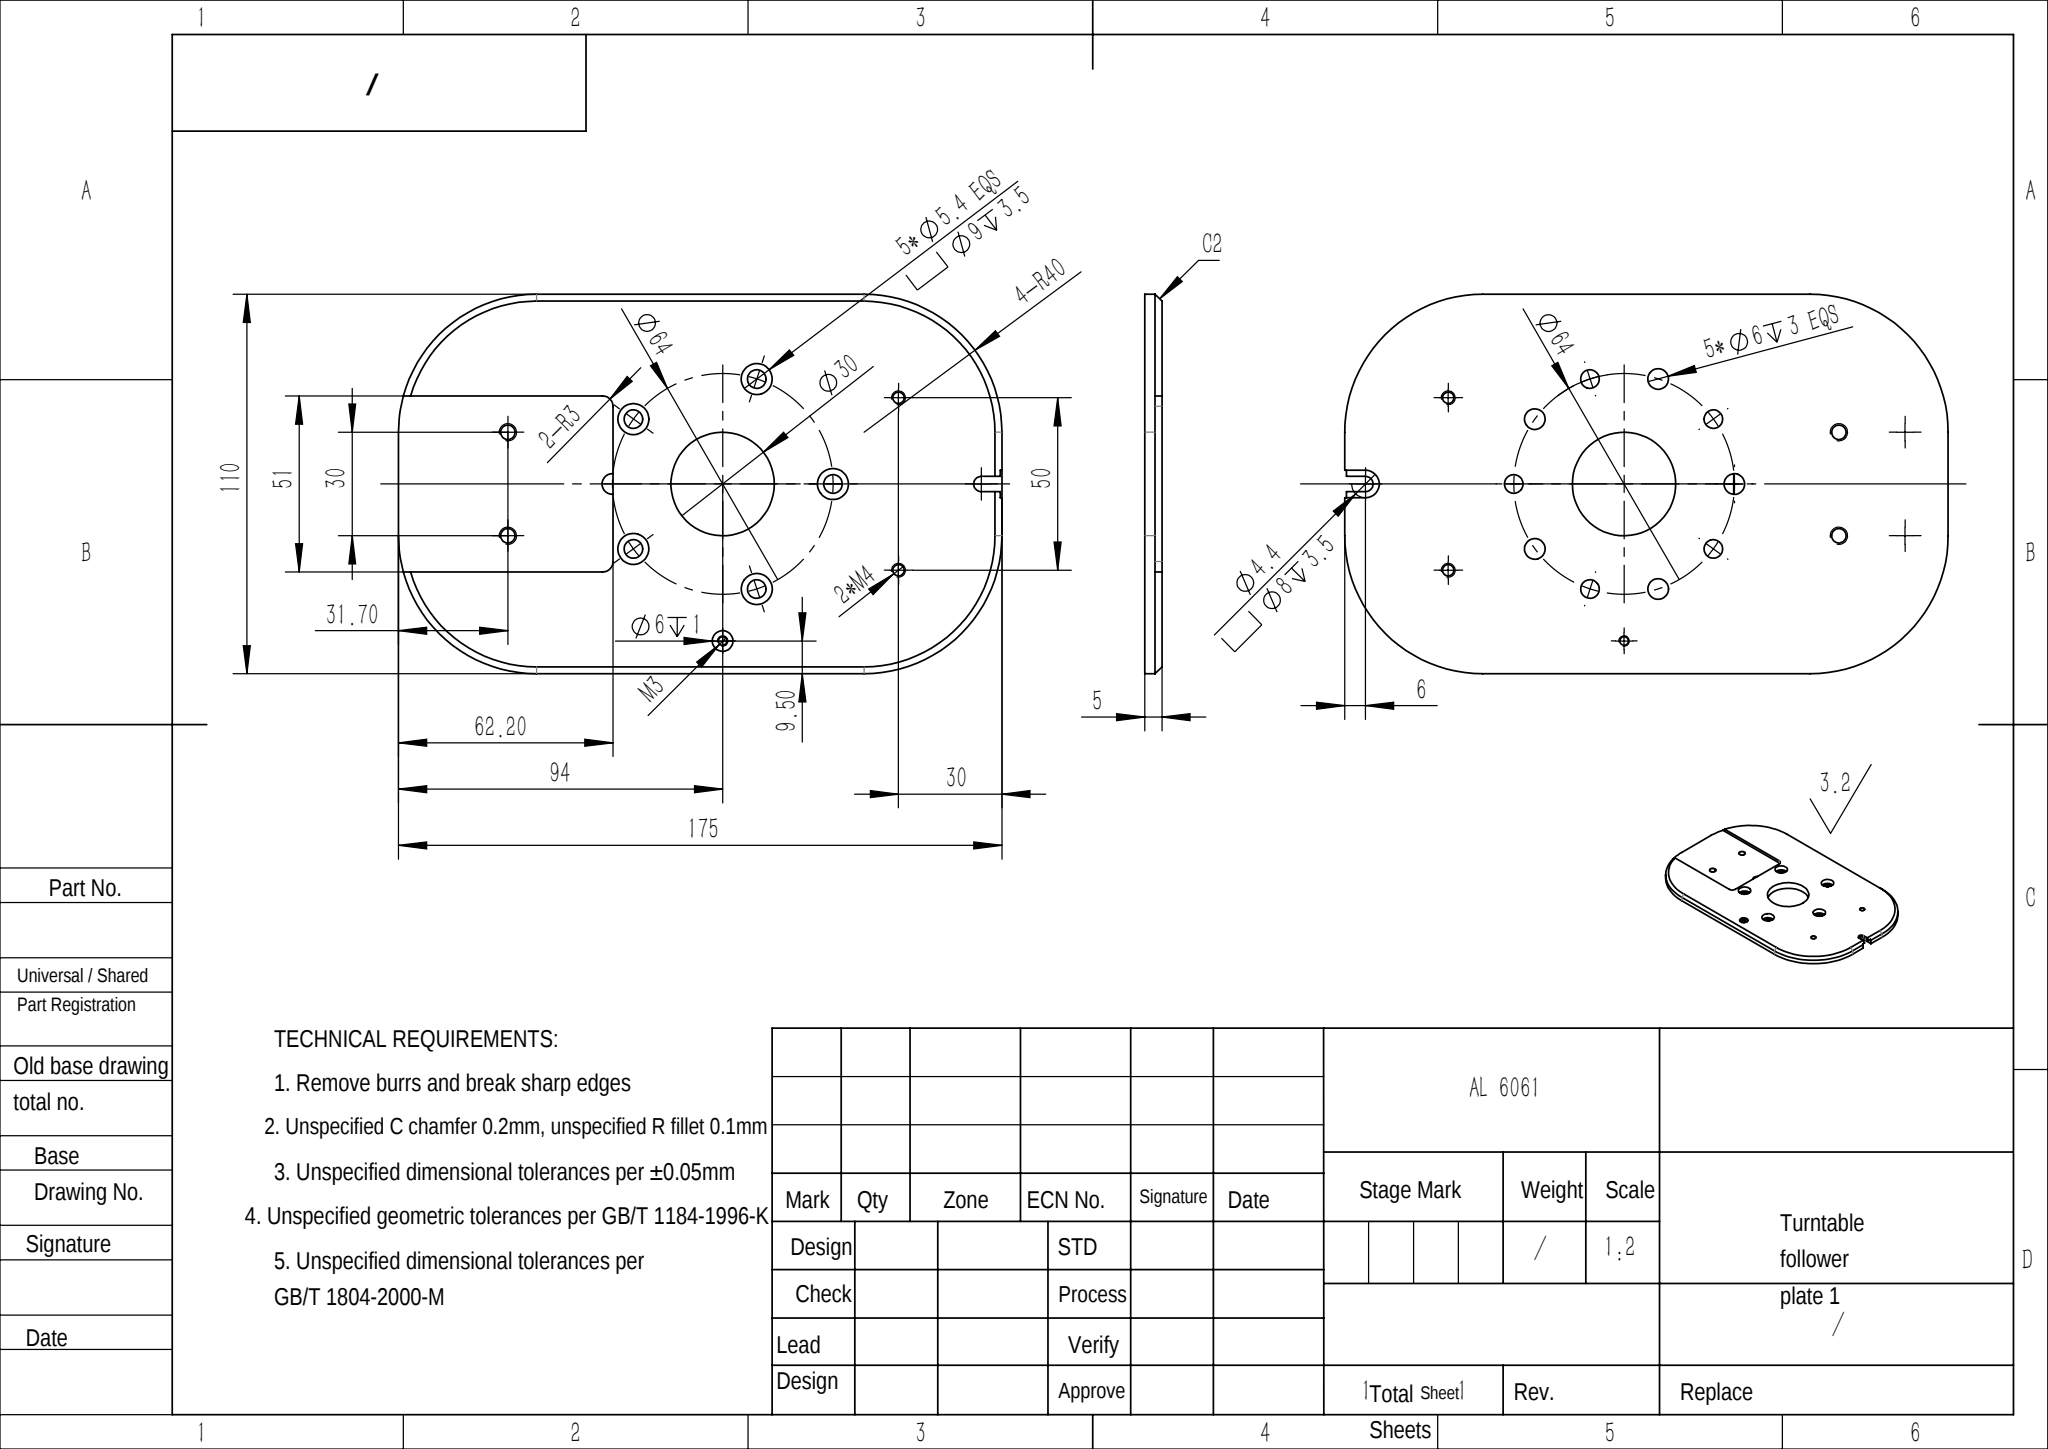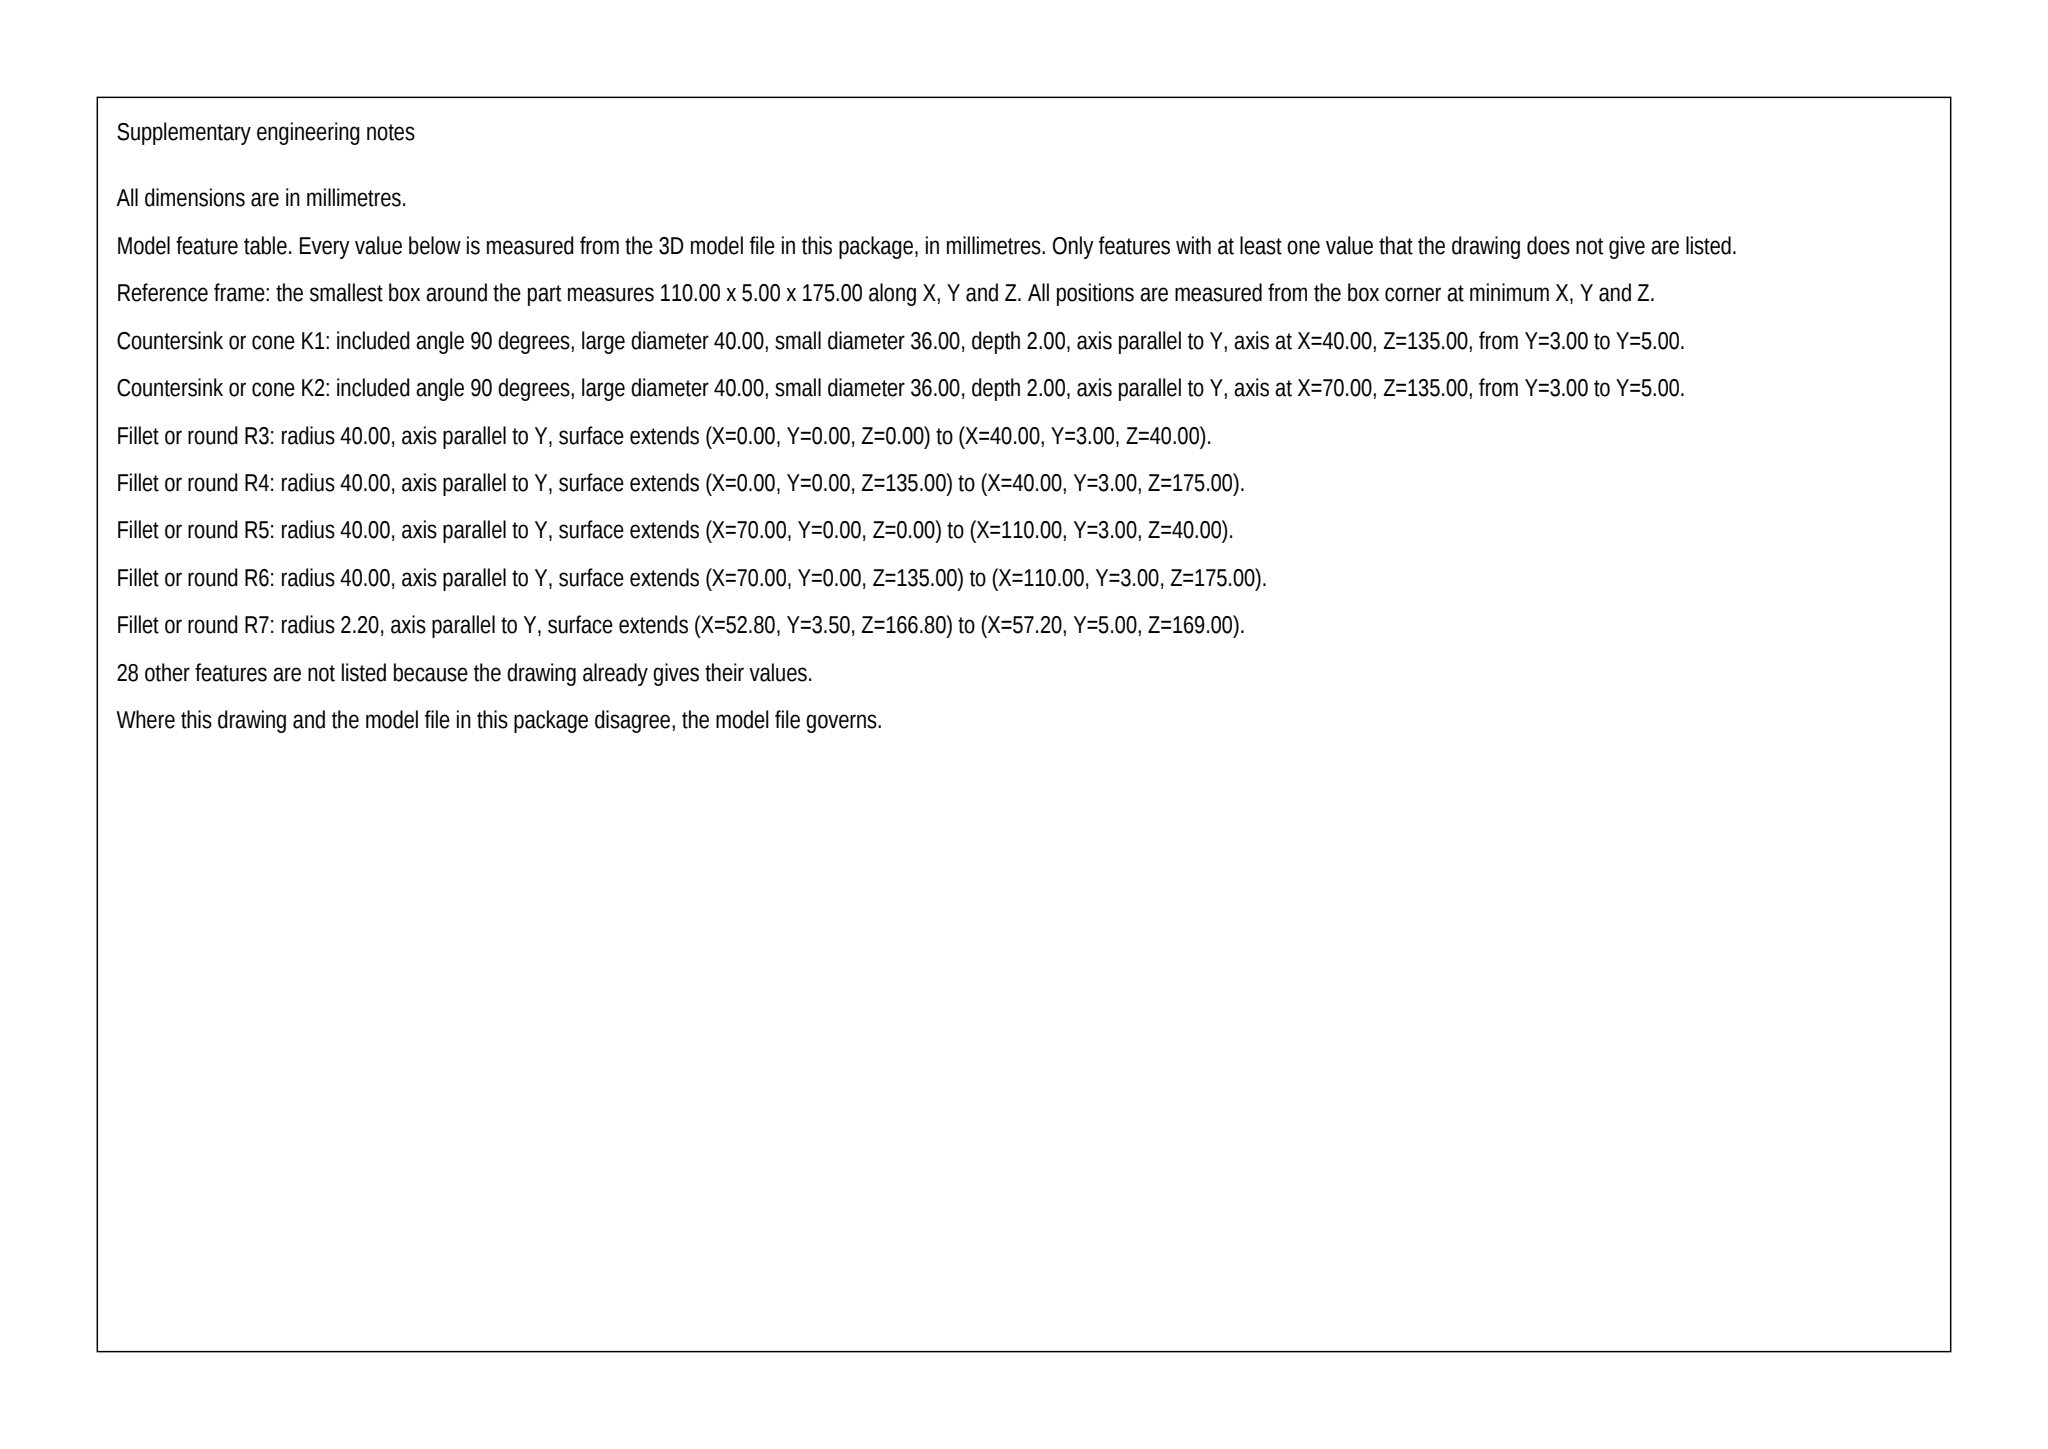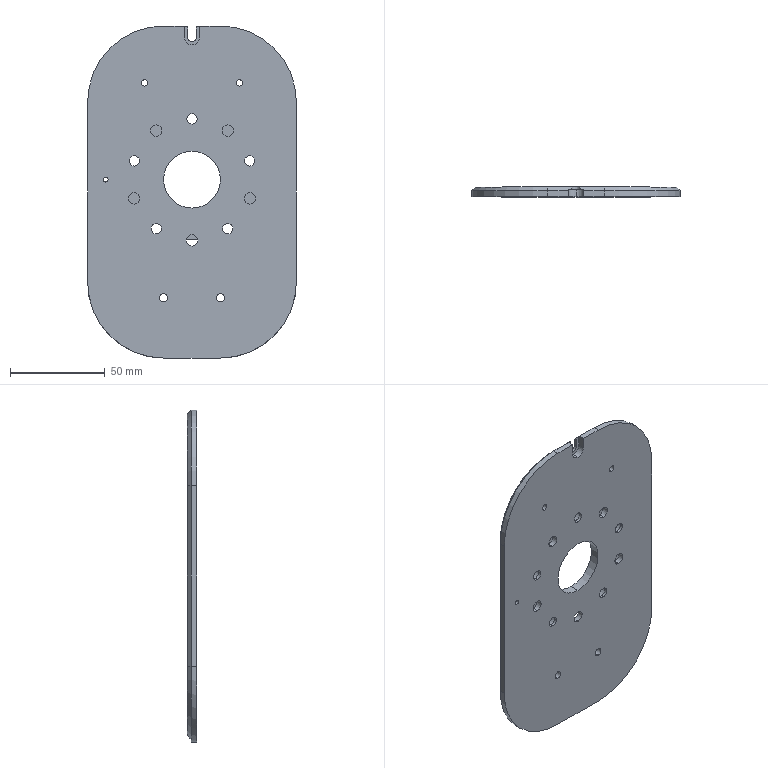Part | SolidWorks | mm | material AL 6061 | 1 solid | 88 faces | box 110 x 5 x 175 mm | volume 76416 mm3 | cylinder 53 | plane 31 | cone 4 | commonest cylinder face diameters 6 x14 9 x10 5.4 x10 4.2 x4 3.3 x4 80 x4 30 x2 2.5 x2